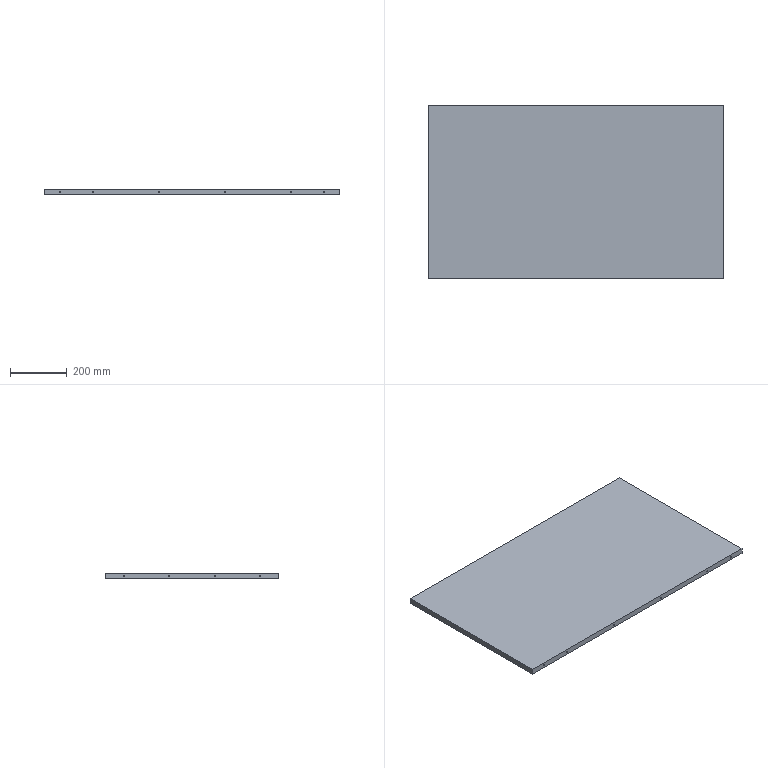Component | NX | TOP_COVER | 1 solid | 31 faces | volume 3416410 mm3 | cylinder 20 | plane 11 | commonest cylinder face diameters 4.5 x20